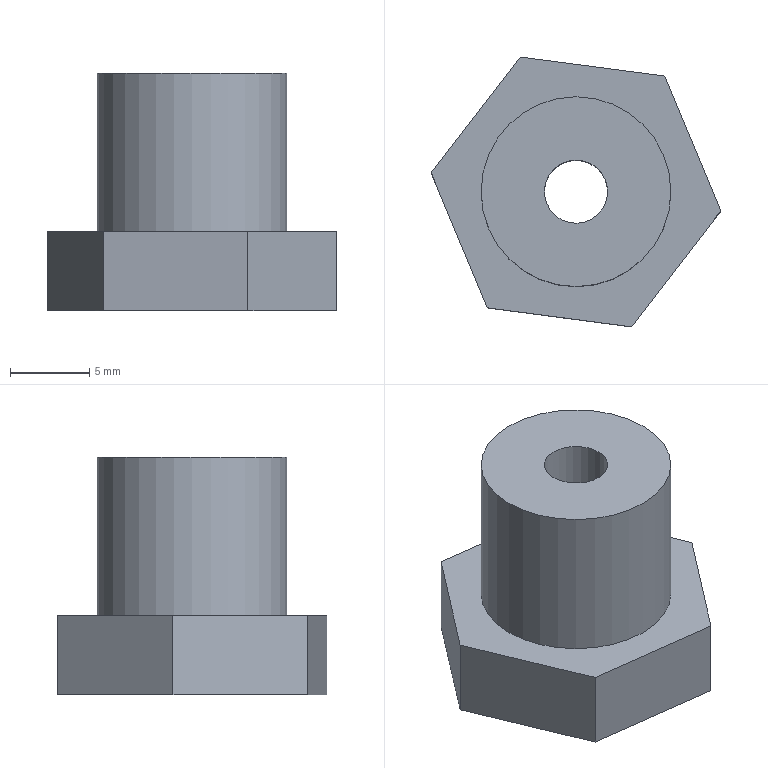Component | NX | 09__27_2 | 1 solid | 11 faces | box 18.32 x 17.07 x 15 mm | volume 2051 mm3 | plane 9 | cylinder 2 | commonest cylinder face diameters 4 x1 12 x1
STEP:
#1=CARTESIAN_POINT('',(0.,0.,0.));
#2=DIRECTION('',(0.,0.,1.));
#3=DIRECTION('',(1.,0.,0.));
#4=AXIS2_PLACEMENT_3D('',#1,#2,#3);
#5=CARTESIAN_POINT('',(70.402,102.259,175.932));
#6=VERTEX_POINT('',#5);
#7=CARTESIAN_POINT('',(66.863,110.792,175.932));
#8=VERTEX_POINT('',#7);
#9=CARTESIAN_POINT('',(70.402,102.259,175.932));
#10=DIRECTION('',(-0.383,0.9237,0.));
#11=VECTOR('',#10,1.);
#12=LINE('',#9,#11);
#13=CARTESIAN_POINT('',(70.402,102.259,170.932));
#14=DIRECTION('',(0.9237,0.383,0.));
#15=DIRECTION('',(0.383,-0.9237,0.));
#16=AXIS2_PLACEMENT_3D('',#13,#14,#15);
#17=PLANE('',#16);
#18=CARTESIAN_POINT('',(0.,-5.));
#19=DIRECTION('',(-1.,0.));
#20=VECTOR('',#19,1.);
#21=LINE('',#18,#20);
#22=(GEOMETRIC_REPRESENTATION_CONTEXT(2)PARAMETRIC_REPRESENTATION_CONTEXT()REPRESENTATION_CONTEXT('',''));
#23=DEFINITIONAL_REPRESENTATION('',(#21),#22);
#24=PCURVE('',#17,#23);
#25=CARTESIAN_POINT('',(76.022,109.59,175.932));
#26=DIRECTION('',(0.,0.,-1.));
#27=DIRECTION('',(0.9237,0.383,0.));
#28=AXIS2_PLACEMENT_3D('',#25,#26,#27);
#29=PLANE('',#28);
#30=CARTESIAN_POINT('',(-8.,4.619));
#31=DIRECTION('',(-0.,-1.));
#32=VECTOR('',#31,1.);
#33=LINE('',#30,#32);
#34=(GEOMETRIC_REPRESENTATION_CONTEXT(2)PARAMETRIC_REPRESENTATION_CONTEXT()REPRESENTATION_CONTEXT('',''));
#35=DEFINITIONAL_REPRESENTATION('',(#33),#34);
#36=PCURVE('',#29,#35);
#37=SURFACE_CURVE('',#12,(#24,#36),.PCURVE_S1.);
#38=EDGE_CURVE('',#6,#8,#37,.T.);
#39=ORIENTED_EDGE('',*,*,#38,.T.);
#40=CARTESIAN_POINT('',(66.863,110.792,170.932));
#41=VERTEX_POINT('',#40);
#42=CARTESIAN_POINT('',(66.863,110.792,170.932));
#43=DIRECTION('',(0.,0.,1.));
#44=VECTOR('',#43,1.);
#45=LINE('',#42,#44);
#46=CARTESIAN_POINT('',(-9.238,0.));
#47=DIRECTION('',(0.,-1.));
#48=VECTOR('',#47,1.);
#49=LINE('',#46,#48);
#50=(GEOMETRIC_REPRESENTATION_CONTEXT(2)PARAMETRIC_REPRESENTATION_CONTEXT()REPRESENTATION_CONTEXT('',''));
#51=DEFINITIONAL_REPRESENTATION('',(#49),#50);
#52=PCURVE('',#17,#51);
#53=CARTESIAN_POINT('',(66.863,110.792,170.932));
#54=DIRECTION('',(0.7936,-0.6084,0.));
#55=DIRECTION('',(-0.6084,-0.7936,0.));
#56=AXIS2_PLACEMENT_3D('',#53,#54,#55);
#57=PLANE('',#56);
#58=CARTESIAN_POINT('',(0.,0.));
#59=DIRECTION('',(0.,-1.));
#60=VECTOR('',#59,1.);
#61=LINE('',#58,#60);
#62=(GEOMETRIC_REPRESENTATION_CONTEXT(2)PARAMETRIC_REPRESENTATION_CONTEXT()REPRESENTATION_CONTEXT('',''));
#63=DEFINITIONAL_REPRESENTATION('',(#61),#62);
#64=PCURVE('',#57,#63);
#65=SURFACE_CURVE('',#45,(#52,#64),.PCURVE_S1.);
#66=EDGE_CURVE('',#41,#8,#65,.T.);
#67=ORIENTED_EDGE('',*,*,#66,.F.);
#68=CARTESIAN_POINT('',(70.402,102.259,170.932));
#69=VERTEX_POINT('',#68);
#70=CARTESIAN_POINT('',(70.402,102.259,170.932));
#71=DIRECTION('',(-0.383,0.9237,0.));
#72=VECTOR('',#71,1.);
#73=LINE('',#70,#72);
#74=CARTESIAN_POINT('',(0.,0.));
#75=DIRECTION('',(-1.,0.));
#76=VECTOR('',#75,1.);
#77=LINE('',#74,#76);
#78=(GEOMETRIC_REPRESENTATION_CONTEXT(2)PARAMETRIC_REPRESENTATION_CONTEXT()REPRESENTATION_CONTEXT('',''));
#79=DEFINITIONAL_REPRESENTATION('',(#77),#78);
#80=PCURVE('',#17,#79);
#81=CARTESIAN_POINT('',(76.022,109.59,170.932));
#82=DIRECTION('',(0.,0.,-1.));
#83=DIRECTION('',(0.9237,0.383,0.));
#84=AXIS2_PLACEMENT_3D('',#81,#82,#83);
#85=PLANE('',#84);
#86=CARTESIAN_POINT('',(-8.,4.619));
#87=DIRECTION('',(-0.,-1.));
#88=VECTOR('',#87,1.);
#89=LINE('',#86,#88);
#90=(GEOMETRIC_REPRESENTATION_CONTEXT(2)PARAMETRIC_REPRESENTATION_CONTEXT()REPRESENTATION_CONTEXT('',''));
#91=DEFINITIONAL_REPRESENTATION('',(#89),#90);
#92=PCURVE('',#85,#91);
#93=SURFACE_CURVE('',#73,(#80,#92),.PCURVE_S1.);
#94=EDGE_CURVE('',#69,#41,#93,.T.);
#95=ORIENTED_EDGE('',*,*,#94,.F.);
#96=CARTESIAN_POINT('',(70.402,102.259,170.932));
#97=DIRECTION('',(0.,0.,1.));
#98=VECTOR('',#97,1.);
#99=LINE('',#96,#98);
#100=CARTESIAN_POINT('',(0.,0.));
#101=DIRECTION('',(0.,-1.));
#102=VECTOR('',#101,1.);
#103=LINE('',#100,#102);
#104=(GEOMETRIC_REPRESENTATION_CONTEXT(2)PARAMETRIC_REPRESENTATION_CONTEXT()REPRESENTATION_CONTEXT('',''));
#105=DEFINITIONAL_REPRESENTATION('',(#103),#104);
#106=PCURVE('',#17,#105);
#107=CARTESIAN_POINT('',(79.561,101.057,170.932));
#108=DIRECTION('',(0.1301,0.9915,0.));
#109=DIRECTION('',(0.9915,-0.1301,0.));
#110=AXIS2_PLACEMENT_3D('',#107,#108,#109);
#111=PLANE('',#110);
#112=CARTESIAN_POINT('',(-9.238,0.));
#113=DIRECTION('',(0.,-1.));
#114=VECTOR('',#113,1.);
#115=LINE('',#112,#114);
#116=(GEOMETRIC_REPRESENTATION_CONTEXT(2)PARAMETRIC_REPRESENTATION_CONTEXT()REPRESENTATION_CONTEXT('',''));
#117=DEFINITIONAL_REPRESENTATION('',(#115),#116);
#118=PCURVE('',#111,#117);
#119=SURFACE_CURVE('',#99,(#106,#118),.PCURVE_S1.);
#120=EDGE_CURVE('',#69,#6,#119,.T.);
#121=ORIENTED_EDGE('',*,*,#120,.T.);
#122=EDGE_LOOP('',(#39,#67,#95,#121));
#123=FACE_BOUND('',#122,.T.);
#124=ADVANCED_FACE('',(#123),#17,.F.);
#125=CARTESIAN_POINT('',(72.484,118.123,175.932));
#126=VERTEX_POINT('',#125);
#127=CARTESIAN_POINT('',(66.863,110.792,175.932));
#128=DIRECTION('',(0.6084,0.7936,0.));
#129=VECTOR('',#128,1.);
#130=LINE('',#127,#129);
#131=CARTESIAN_POINT('',(0.,-5.));
#132=DIRECTION('',(-1.,0.));
#133=VECTOR('',#132,1.);
#134=LINE('',#131,#133);
#135=(GEOMETRIC_REPRESENTATION_CONTEXT(2)PARAMETRIC_REPRESENTATION_CONTEXT()REPRESENTATION_CONTEXT('',''));
#136=DEFINITIONAL_REPRESENTATION('',(#134),#135);
#137=PCURVE('',#57,#136);
#138=CARTESIAN_POINT('',(-8.,-4.619));
#139=DIRECTION('',(0.866,-0.5));
#140=VECTOR('',#139,1.);
#141=LINE('',#138,#140);
#142=(GEOMETRIC_REPRESENTATION_CONTEXT(2)PARAMETRIC_REPRESENTATION_CONTEXT()REPRESENTATION_CONTEXT('',''));
#143=DEFINITIONAL_REPRESENTATION('',(#141),#142);
#144=PCURVE('',#29,#143);
#145=SURFACE_CURVE('',#130,(#137,#144),.PCURVE_S1.);
#146=EDGE_CURVE('',#8,#126,#145,.T.);
#147=ORIENTED_EDGE('',*,*,#146,.T.);
#148=CARTESIAN_POINT('',(72.484,118.123,170.932));
#149=VERTEX_POINT('',#148);
#150=CARTESIAN_POINT('',(72.484,118.123,170.932));
#151=DIRECTION('',(0.,0.,1.));
#152=VECTOR('',#151,1.);
#153=LINE('',#150,#152);
#154=CARTESIAN_POINT('',(-9.238,0.));
#155=DIRECTION('',(0.,-1.));
#156=VECTOR('',#155,1.);
#157=LINE('',#154,#156);
#158=(GEOMETRIC_REPRESENTATION_CONTEXT(2)PARAMETRIC_REPRESENTATION_CONTEXT()REPRESENTATION_CONTEXT('',''));
#159=DEFINITIONAL_REPRESENTATION('',(#157),#158);
#160=PCURVE('',#57,#159);
#161=CARTESIAN_POINT('',(72.484,118.123,170.932));
#162=DIRECTION('',(-0.1301,-0.9915,0.));
#163=DIRECTION('',(-0.9915,0.1301,0.));
#164=AXIS2_PLACEMENT_3D('',#161,#162,#163);
#165=PLANE('',#164);
#166=CARTESIAN_POINT('',(0.,0.));
#167=DIRECTION('',(0.,-1.));
#168=VECTOR('',#167,1.);
#169=LINE('',#166,#168);
#170=(GEOMETRIC_REPRESENTATION_CONTEXT(2)PARAMETRIC_REPRESENTATION_CONTEXT()REPRESENTATION_CONTEXT('',''));
#171=DEFINITIONAL_REPRESENTATION('',(#169),#170);
#172=PCURVE('',#165,#171);
#173=SURFACE_CURVE('',#153,(#160,#172),.PCURVE_S1.);
#174=EDGE_CURVE('',#149,#126,#173,.T.);
#175=ORIENTED_EDGE('',*,*,#174,.F.);
#176=CARTESIAN_POINT('',(66.863,110.792,170.932));
#177=DIRECTION('',(0.6084,0.7936,0.));
#178=VECTOR('',#177,1.);
#179=LINE('',#176,#178);
#180=CARTESIAN_POINT('',(0.,0.));
#181=DIRECTION('',(-1.,0.));
#182=VECTOR('',#181,1.);
#183=LINE('',#180,#182);
#184=(GEOMETRIC_REPRESENTATION_CONTEXT(2)PARAMETRIC_REPRESENTATION_CONTEXT()REPRESENTATION_CONTEXT('',''));
#185=DEFINITIONAL_REPRESENTATION('',(#183),#184);
#186=PCURVE('',#57,#185);
#187=CARTESIAN_POINT('',(-8.,-4.619));
#188=DIRECTION('',(0.866,-0.5));
#189=VECTOR('',#188,1.);
#190=LINE('',#187,#189);
#191=(GEOMETRIC_REPRESENTATION_CONTEXT(2)PARAMETRIC_REPRESENTATION_CONTEXT()REPRESENTATION_CONTEXT('',''));
#192=DEFINITIONAL_REPRESENTATION('',(#190),#191);
#193=PCURVE('',#85,#192);
#194=SURFACE_CURVE('',#179,(#186,#193),.PCURVE_S1.);
#195=EDGE_CURVE('',#41,#149,#194,.T.);
#196=ORIENTED_EDGE('',*,*,#195,.F.);
#197=ORIENTED_EDGE('',*,*,#66,.T.);
#198=EDGE_LOOP('',(#147,#175,#196,#197));
#199=FACE_BOUND('',#198,.T.);
#200=ADVANCED_FACE('',(#199),#57,.F.);
#201=CARTESIAN_POINT('',(81.643,116.921,175.932));
#202=VERTEX_POINT('',#201);
#203=CARTESIAN_POINT('',(72.484,118.123,175.932));
#204=DIRECTION('',(0.9915,-0.1301,0.));
#205=VECTOR('',#204,1.);
#206=LINE('',#203,#205);
#207=CARTESIAN_POINT('',(0.,-5.));
#208=DIRECTION('',(-1.,0.));
#209=VECTOR('',#208,1.);
#210=LINE('',#207,#209);
#211=(GEOMETRIC_REPRESENTATION_CONTEXT(2)PARAMETRIC_REPRESENTATION_CONTEXT()REPRESENTATION_CONTEXT('',''));
#212=DEFINITIONAL_REPRESENTATION('',(#210),#211);
#213=PCURVE('',#165,#212);
#214=CARTESIAN_POINT('',(0.,-9.238));
#215=DIRECTION('',(0.866,0.5));
#216=VECTOR('',#215,1.);
#217=LINE('',#214,#216);
#218=(GEOMETRIC_REPRESENTATION_CONTEXT(2)PARAMETRIC_REPRESENTATION_CONTEXT()REPRESENTATION_CONTEXT('',''));
#219=DEFINITIONAL_REPRESENTATION('',(#217),#218);
#220=PCURVE('',#29,#219);
#221=SURFACE_CURVE('',#206,(#213,#220),.PCURVE_S1.);
#222=EDGE_CURVE('',#126,#202,#221,.T.);
#223=ORIENTED_EDGE('',*,*,#222,.T.);
#224=CARTESIAN_POINT('',(81.643,116.921,170.932));
#225=VERTEX_POINT('',#224);
#226=CARTESIAN_POINT('',(81.643,116.921,170.932));
#227=DIRECTION('',(0.,0.,1.));
#228=VECTOR('',#227,1.);
#229=LINE('',#226,#228);
#230=CARTESIAN_POINT('',(-9.238,0.));
#231=DIRECTION('',(0.,-1.));
#232=VECTOR('',#231,1.);
#233=LINE('',#230,#232);
#234=(GEOMETRIC_REPRESENTATION_CONTEXT(2)PARAMETRIC_REPRESENTATION_CONTEXT()REPRESENTATION_CONTEXT('',''));
#235=DEFINITIONAL_REPRESENTATION('',(#233),#234);
#236=PCURVE('',#165,#235);
#237=CARTESIAN_POINT('',(81.643,116.921,170.932));
#238=DIRECTION('',(-0.9237,-0.383,0.));
#239=DIRECTION('',(-0.383,0.9237,0.));
#240=AXIS2_PLACEMENT_3D('',#237,#238,#239);
#241=PLANE('',#240);
#242=CARTESIAN_POINT('',(0.,0.));
#243=DIRECTION('',(0.,-1.));
#244=VECTOR('',#243,1.);
#245=LINE('',#242,#244);
#246=(GEOMETRIC_REPRESENTATION_CONTEXT(2)PARAMETRIC_REPRESENTATION_CONTEXT()REPRESENTATION_CONTEXT('',''));
#247=DEFINITIONAL_REPRESENTATION('',(#245),#246);
#248=PCURVE('',#241,#247);
#249=SURFACE_CURVE('',#229,(#236,#248),.PCURVE_S1.);
#250=EDGE_CURVE('',#225,#202,#249,.T.);
#251=ORIENTED_EDGE('',*,*,#250,.F.);
#252=CARTESIAN_POINT('',(72.484,118.123,170.932));
#253=DIRECTION('',(0.9915,-0.1301,0.));
#254=VECTOR('',#253,1.);
#255=LINE('',#252,#254);
#256=CARTESIAN_POINT('',(0.,0.));
#257=DIRECTION('',(-1.,0.));
#258=VECTOR('',#257,1.);
#259=LINE('',#256,#258);
#260=(GEOMETRIC_REPRESENTATION_CONTEXT(2)PARAMETRIC_REPRESENTATION_CONTEXT()REPRESENTATION_CONTEXT('',''));
#261=DEFINITIONAL_REPRESENTATION('',(#259),#260);
#262=PCURVE('',#165,#261);
#263=CARTESIAN_POINT('',(0.,-9.238));
#264=DIRECTION('',(0.866,0.5));
#265=VECTOR('',#264,1.);
#266=LINE('',#263,#265);
#267=(GEOMETRIC_REPRESENTATION_CONTEXT(2)PARAMETRIC_REPRESENTATION_CONTEXT()REPRESENTATION_CONTEXT('',''));
#268=DEFINITIONAL_REPRESENTATION('',(#266),#267);
#269=PCURVE('',#85,#268);
#270=SURFACE_CURVE('',#255,(#262,#269),.PCURVE_S1.);
#271=EDGE_CURVE('',#149,#225,#270,.T.);
#272=ORIENTED_EDGE('',*,*,#271,.F.);
#273=ORIENTED_EDGE('',*,*,#174,.T.);
#274=EDGE_LOOP('',(#223,#251,#272,#273));
#275=FACE_BOUND('',#274,.T.);
#276=ADVANCED_FACE('',(#275),#165,.F.);
#277=CARTESIAN_POINT('',(85.181,108.388,175.932));
#278=VERTEX_POINT('',#277);
#279=CARTESIAN_POINT('',(81.643,116.921,175.932));
#280=DIRECTION('',(0.383,-0.9237,0.));
#281=VECTOR('',#280,1.);
#282=LINE('',#279,#281);
#283=CARTESIAN_POINT('',(0.,-5.));
#284=DIRECTION('',(-1.,0.));
#285=VECTOR('',#284,1.);
#286=LINE('',#283,#285);
#287=(GEOMETRIC_REPRESENTATION_CONTEXT(2)PARAMETRIC_REPRESENTATION_CONTEXT()REPRESENTATION_CONTEXT('',''));
#288=DEFINITIONAL_REPRESENTATION('',(#286),#287);
#289=PCURVE('',#241,#288);
#290=CARTESIAN_POINT('',(8.,-4.619));
#291=DIRECTION('',(0.,1.));
#292=VECTOR('',#291,1.);
#293=LINE('',#290,#292);
#294=(GEOMETRIC_REPRESENTATION_CONTEXT(2)PARAMETRIC_REPRESENTATION_CONTEXT()REPRESENTATION_CONTEXT('',''));
#295=DEFINITIONAL_REPRESENTATION('',(#293),#294);
#296=PCURVE('',#29,#295);
#297=SURFACE_CURVE('',#282,(#289,#296),.PCURVE_S1.);
#298=EDGE_CURVE('',#202,#278,#297,.T.);
#299=ORIENTED_EDGE('',*,*,#298,.T.);
#300=CARTESIAN_POINT('',(85.181,108.388,170.932));
#301=VERTEX_POINT('',#300);
#302=CARTESIAN_POINT('',(85.181,108.388,170.932));
#303=DIRECTION('',(0.,0.,1.));
#304=VECTOR('',#303,1.);
#305=LINE('',#302,#304);
#306=CARTESIAN_POINT('',(-9.238,0.));
#307=DIRECTION('',(0.,-1.));
#308=VECTOR('',#307,1.);
#309=LINE('',#306,#308);
#310=(GEOMETRIC_REPRESENTATION_CONTEXT(2)PARAMETRIC_REPRESENTATION_CONTEXT()REPRESENTATION_CONTEXT('',''));
#311=DEFINITIONAL_REPRESENTATION('',(#309),#310);
#312=PCURVE('',#241,#311);
#313=CARTESIAN_POINT('',(85.181,108.388,170.932));
#314=DIRECTION('',(-0.7936,0.6084,0.));
#315=DIRECTION('',(0.6084,0.7936,0.));
#316=AXIS2_PLACEMENT_3D('',#313,#314,#315);
#317=PLANE('',#316);
#318=CARTESIAN_POINT('',(0.,0.));
#319=DIRECTION('',(0.,-1.));
#320=VECTOR('',#319,1.);
#321=LINE('',#318,#320);
#322=(GEOMETRIC_REPRESENTATION_CONTEXT(2)PARAMETRIC_REPRESENTATION_CONTEXT()REPRESENTATION_CONTEXT('',''));
#323=DEFINITIONAL_REPRESENTATION('',(#321),#322);
#324=PCURVE('',#317,#323);
#325=SURFACE_CURVE('',#305,(#312,#324),.PCURVE_S1.);
#326=EDGE_CURVE('',#301,#278,#325,.T.);
#327=ORIENTED_EDGE('',*,*,#326,.F.);
#328=CARTESIAN_POINT('',(81.643,116.921,170.932));
#329=DIRECTION('',(0.383,-0.9237,0.));
#330=VECTOR('',#329,1.);
#331=LINE('',#328,#330);
#332=CARTESIAN_POINT('',(0.,0.));
#333=DIRECTION('',(-1.,0.));
#334=VECTOR('',#333,1.);
#335=LINE('',#332,#334);
#336=(GEOMETRIC_REPRESENTATION_CONTEXT(2)PARAMETRIC_REPRESENTATION_CONTEXT()REPRESENTATION_CONTEXT('',''));
#337=DEFINITIONAL_REPRESENTATION('',(#335),#336);
#338=PCURVE('',#241,#337);
#339=CARTESIAN_POINT('',(8.,-4.619));
#340=DIRECTION('',(0.,1.));
#341=VECTOR('',#340,1.);
#342=LINE('',#339,#341);
#343=(GEOMETRIC_REPRESENTATION_CONTEXT(2)PARAMETRIC_REPRESENTATION_CONTEXT()REPRESENTATION_CONTEXT('',''));
#344=DEFINITIONAL_REPRESENTATION('',(#342),#343);
#345=PCURVE('',#85,#344);
#346=SURFACE_CURVE('',#331,(#338,#345),.PCURVE_S1.);
#347=EDGE_CURVE('',#225,#301,#346,.T.);
#348=ORIENTED_EDGE('',*,*,#347,.F.);
#349=ORIENTED_EDGE('',*,*,#250,.T.);
#350=EDGE_LOOP('',(#299,#327,#348,#349));
#351=FACE_BOUND('',#350,.T.);
#352=ADVANCED_FACE('',(#351),#241,.F.);
#353=CARTESIAN_POINT('',(79.561,101.057,175.932));
#354=VERTEX_POINT('',#353);
#355=CARTESIAN_POINT('',(85.181,108.388,175.932));
#356=DIRECTION('',(-0.6084,-0.7936,0.));
#357=VECTOR('',#356,1.);
#358=LINE('',#355,#357);
#359=CARTESIAN_POINT('',(0.,-5.));
#360=DIRECTION('',(-1.,0.));
#361=VECTOR('',#360,1.);
#362=LINE('',#359,#361);
#363=(GEOMETRIC_REPRESENTATION_CONTEXT(2)PARAMETRIC_REPRESENTATION_CONTEXT()REPRESENTATION_CONTEXT('',''));
#364=DEFINITIONAL_REPRESENTATION('',(#362),#363);
#365=PCURVE('',#317,#364);
#366=CARTESIAN_POINT('',(8.,4.619));
#367=DIRECTION('',(-0.866,0.5));
#368=VECTOR('',#367,1.);
#369=LINE('',#366,#368);
#370=(GEOMETRIC_REPRESENTATION_CONTEXT(2)PARAMETRIC_REPRESENTATION_CONTEXT()REPRESENTATION_CONTEXT('',''));
#371=DEFINITIONAL_REPRESENTATION('',(#369),#370);
#372=PCURVE('',#29,#371);
#373=SURFACE_CURVE('',#358,(#365,#372),.PCURVE_S1.);
#374=EDGE_CURVE('',#278,#354,#373,.T.);
#375=ORIENTED_EDGE('',*,*,#374,.T.);
#376=CARTESIAN_POINT('',(79.561,101.057,170.932));
#377=VERTEX_POINT('',#376);
#378=CARTESIAN_POINT('',(79.561,101.057,170.932));
#379=DIRECTION('',(0.,0.,1.));
#380=VECTOR('',#379,1.);
#381=LINE('',#378,#380);
#382=CARTESIAN_POINT('',(-9.238,0.));
#383=DIRECTION('',(0.,-1.));
#384=VECTOR('',#383,1.);
#385=LINE('',#382,#384);
#386=(GEOMETRIC_REPRESENTATION_CONTEXT(2)PARAMETRIC_REPRESENTATION_CONTEXT()REPRESENTATION_CONTEXT('',''));
#387=DEFINITIONAL_REPRESENTATION('',(#385),#386);
#388=PCURVE('',#317,#387);
#389=CARTESIAN_POINT('',(0.,0.));
#390=DIRECTION('',(0.,-1.));
#391=VECTOR('',#390,1.);
#392=LINE('',#389,#391);
#393=(GEOMETRIC_REPRESENTATION_CONTEXT(2)PARAMETRIC_REPRESENTATION_CONTEXT()REPRESENTATION_CONTEXT('',''));
#394=DEFINITIONAL_REPRESENTATION('',(#392),#393);
#395=PCURVE('',#111,#394);
#396=SURFACE_CURVE('',#381,(#388,#395),.PCURVE_S1.);
#397=EDGE_CURVE('',#377,#354,#396,.T.);
#398=ORIENTED_EDGE('',*,*,#397,.F.);
#399=CARTESIAN_POINT('',(85.181,108.388,170.932));
#400=DIRECTION('',(-0.6084,-0.7936,0.));
#401=VECTOR('',#400,1.);
#402=LINE('',#399,#401);
#403=CARTESIAN_POINT('',(0.,0.));
#404=DIRECTION('',(-1.,0.));
#405=VECTOR('',#404,1.);
#406=LINE('',#403,#405);
#407=(GEOMETRIC_REPRESENTATION_CONTEXT(2)PARAMETRIC_REPRESENTATION_CONTEXT()REPRESENTATION_CONTEXT('',''));
#408=DEFINITIONAL_REPRESENTATION('',(#406),#407);
#409=PCURVE('',#317,#408);
#410=CARTESIAN_POINT('',(8.,4.619));
#411=DIRECTION('',(-0.866,0.5));
#412=VECTOR('',#411,1.);
#413=LINE('',#410,#412);
#414=(GEOMETRIC_REPRESENTATION_CONTEXT(2)PARAMETRIC_REPRESENTATION_CONTEXT()REPRESENTATION_CONTEXT('',''));
#415=DEFINITIONAL_REPRESENTATION('',(#413),#414);
#416=PCURVE('',#85,#415);
#417=SURFACE_CURVE('',#402,(#409,#416),.PCURVE_S1.);
#418=EDGE_CURVE('',#301,#377,#417,.T.);
#419=ORIENTED_EDGE('',*,*,#418,.F.);
#420=ORIENTED_EDGE('',*,*,#326,.T.);
#421=EDGE_LOOP('',(#375,#398,#419,#420));
#422=FACE_BOUND('',#421,.T.);
#423=ADVANCED_FACE('',(#422),#317,.F.);
#424=CARTESIAN_POINT('',(79.561,101.057,175.932));
#425=DIRECTION('',(-0.9915,0.1301,0.));
#426=VECTOR('',#425,1.);
#427=LINE('',#424,#426);
#428=CARTESIAN_POINT('',(0.,-5.));
#429=DIRECTION('',(-1.,0.));
#430=VECTOR('',#429,1.);
#431=LINE('',#428,#430);
#432=(GEOMETRIC_REPRESENTATION_CONTEXT(2)PARAMETRIC_REPRESENTATION_CONTEXT()REPRESENTATION_CONTEXT('',''));
#433=DEFINITIONAL_REPRESENTATION('',(#431),#432);
#434=PCURVE('',#111,#433);
#435=CARTESIAN_POINT('',(-0.,9.238));
#436=DIRECTION('',(-0.866,-0.5));
#437=VECTOR('',#436,1.);
#438=LINE('',#435,#437);
#439=(GEOMETRIC_REPRESENTATION_CONTEXT(2)PARAMETRIC_REPRESENTATION_CONTEXT()REPRESENTATION_CONTEXT('',''));
#440=DEFINITIONAL_REPRESENTATION('',(#438),#439);
#441=PCURVE('',#29,#440);
#442=SURFACE_CURVE('',#427,(#434,#441),.PCURVE_S1.);
#443=EDGE_CURVE('',#354,#6,#442,.T.);
#444=ORIENTED_EDGE('',*,*,#443,.T.);
#445=ORIENTED_EDGE('',*,*,#120,.F.);
#446=CARTESIAN_POINT('',(79.561,101.057,170.932));
#447=DIRECTION('',(-0.9915,0.1301,0.));
#448=VECTOR('',#447,1.);
#449=LINE('',#446,#448);
#450=CARTESIAN_POINT('',(0.,0.));
#451=DIRECTION('',(-1.,0.));
#452=VECTOR('',#451,1.);
#453=LINE('',#450,#452);
#454=(GEOMETRIC_REPRESENTATION_CONTEXT(2)PARAMETRIC_REPRESENTATION_CONTEXT()REPRESENTATION_CONTEXT('',''));
#455=DEFINITIONAL_REPRESENTATION('',(#453),#454);
#456=PCURVE('',#111,#455);
#457=CARTESIAN_POINT('',(-0.,9.238));
#458=DIRECTION('',(-0.866,-0.5));
#459=VECTOR('',#458,1.);
#460=LINE('',#457,#459);
#461=(GEOMETRIC_REPRESENTATION_CONTEXT(2)PARAMETRIC_REPRESENTATION_CONTEXT()REPRESENTATION_CONTEXT('',''));
#462=DEFINITIONAL_REPRESENTATION('',(#460),#461);
#463=PCURVE('',#85,#462);
#464=SURFACE_CURVE('',#449,(#456,#463),.PCURVE_S1.);
#465=EDGE_CURVE('',#377,#69,#464,.T.);
#466=ORIENTED_EDGE('',*,*,#465,.F.);
#467=ORIENTED_EDGE('',*,*,#397,.T.);
#468=EDGE_LOOP('',(#444,#445,#466,#467));
#469=FACE_BOUND('',#468,.T.);
#470=ADVANCED_FACE('',(#469),#111,.F.);
#471=CARTESIAN_POINT('',(77.87,110.356,170.932));
#472=VERTEX_POINT('',#471);
#473=CARTESIAN_POINT('',(76.022,109.59,170.932));
#474=DIRECTION('',(0.,0.,-1.));
#475=DIRECTION('',(0.9237,0.383,0.));
#476=AXIS2_PLACEMENT_3D('',#473,#474,#475);
#477=CIRCLE('',#476,2.);
#478=CARTESIAN_POINT('',(76.022,109.59,170.932));
#479=DIRECTION('',(0.,0.,1.));
#480=DIRECTION('',(-0.9237,-0.383,0.));
#481=AXIS2_PLACEMENT_3D('',#478,#479,#480);
#482=CYLINDRICAL_SURFACE('',#481,2.);
#483=CARTESIAN_POINT('',(9.425,0.));
#484=DIRECTION('',(-1.,0.));
#485=VECTOR('',#484,1.);
#486=LINE('',#483,#485);
#487=(GEOMETRIC_REPRESENTATION_CONTEXT(2)PARAMETRIC_REPRESENTATION_CONTEXT()REPRESENTATION_CONTEXT('',''));
#488=DEFINITIONAL_REPRESENTATION('',(#486),#487);
#489=PCURVE('',#482,#488);
#490=CARTESIAN_POINT('',(0.,0.));
#491=DIRECTION('',(1.,-0.));
#492=AXIS2_PLACEMENT_2D('',#490,#491);
#493=CIRCLE('',#492,2.);
#494=(GEOMETRIC_REPRESENTATION_CONTEXT(2)PARAMETRIC_REPRESENTATION_CONTEXT()REPRESENTATION_CONTEXT('',''));
#495=DEFINITIONAL_REPRESENTATION('',(#493),#494);
#496=PCURVE('',#85,#495);
#497=SURFACE_CURVE('',#477,(#489,#496),.PCURVE_S1.);
#498=EDGE_CURVE('',#472,#472,#497,.T.);
#499=ORIENTED_EDGE('',*,*,#498,.F.);
#500=CARTESIAN_POINT('',(77.87,110.356,185.932));
#501=VERTEX_POINT('',#500);
#502=CARTESIAN_POINT('',(77.87,110.356,170.932));
#503=CARTESIAN_POINT('',(77.87,110.356,185.932));
#504=B_SPLINE_CURVE_WITH_KNOTS('',1,(#502,#503),.UNSPECIFIED.,.F.,.F.,(2,2),(0.,15.),.PIECEWISE_BEZIER_KNOTS.);
#505=CARTESIAN_POINT('',(9.425,0.));
#506=DIRECTION('',(0.,1.));
#507=VECTOR('',#506,1.);
#508=LINE('',#505,#507);
#509=(GEOMETRIC_REPRESENTATION_CONTEXT(2)PARAMETRIC_REPRESENTATION_CONTEXT()REPRESENTATION_CONTEXT('',''));
#510=DEFINITIONAL_REPRESENTATION('',(#508),#509);
#511=PCURVE('',#482,#510);
#512=CARTESIAN_POINT('',(3.142,0.));
#513=DIRECTION('',(0.,1.));
#514=VECTOR('',#513,1.);
#515=LINE('',#512,#514);
#516=(GEOMETRIC_REPRESENTATION_CONTEXT(2)PARAMETRIC_REPRESENTATION_CONTEXT()REPRESENTATION_CONTEXT('',''));
#517=DEFINITIONAL_REPRESENTATION('',(#515),#516);
#518=PCURVE('',#482,#517);
#519=SEAM_CURVE('',#504,(#511,#518),.PCURVE_S1.);
#520=EDGE_CURVE('',#472,#501,#519,.T.);
#521=ORIENTED_EDGE('',*,*,#520,.T.);
#522=CARTESIAN_POINT('',(76.022,109.59,185.932));
#523=DIRECTION('',(0.,0.,-1.));
#524=DIRECTION('',(0.9237,0.383,0.));
#525=AXIS2_PLACEMENT_3D('',#522,#523,#524);
#526=CIRCLE('',#525,2.);
#527=CARTESIAN_POINT('',(9.425,15.));
#528=DIRECTION('',(-1.,0.));
#529=VECTOR('',#528,1.);
#530=LINE('',#527,#529);
#531=(GEOMETRIC_REPRESENTATION_CONTEXT(2)PARAMETRIC_REPRESENTATION_CONTEXT()REPRESENTATION_CONTEXT('',''));
#532=DEFINITIONAL_REPRESENTATION('',(#530),#531);
#533=PCURVE('',#482,#532);
#534=CARTESIAN_POINT('',(76.022,109.59,185.932));
#535=DIRECTION('',(0.,0.,-1.));
#536=DIRECTION('',(0.9237,0.383,0.));
#537=AXIS2_PLACEMENT_3D('',#534,#535,#536);
#538=PLANE('',#537);
#539=CARTESIAN_POINT('',(0.,0.));
#540=DIRECTION('',(1.,-0.));
#541=AXIS2_PLACEMENT_2D('',#539,#540);
#542=CIRCLE('',#541,2.);
#543=(GEOMETRIC_REPRESENTATION_CONTEXT(2)PARAMETRIC_REPRESENTATION_CONTEXT()REPRESENTATION_CONTEXT('',''));
#544=DEFINITIONAL_REPRESENTATION('',(#542),#543);
#545=PCURVE('',#538,#544);
#546=SURFACE_CURVE('',#526,(#533,#545),.PCURVE_S1.);
#547=EDGE_CURVE('',#501,#501,#546,.T.);
#548=ORIENTED_EDGE('',*,*,#547,.T.);
#549=ORIENTED_EDGE('',*,*,#520,.F.);
#550=EDGE_LOOP('',(#499,#521,#548,#549));
#551=FACE_BOUND('',#550,.F.);
#552=ADVANCED_FACE('',(#551),#482,.F.);
#553=ORIENTED_EDGE('',*,*,#94,.T.);
#554=ORIENTED_EDGE('',*,*,#195,.T.);
#555=ORIENTED_EDGE('',*,*,#271,.T.);
#556=ORIENTED_EDGE('',*,*,#347,.T.);
#557=ORIENTED_EDGE('',*,*,#418,.T.);
#558=ORIENTED_EDGE('',*,*,#465,.T.);
#559=EDGE_LOOP('',(#553,#554,#555,#556,#557,#558));
#560=FACE_BOUND('',#559,.T.);
#561=ORIENTED_EDGE('',*,*,#498,.F.);
#562=EDGE_LOOP('',(#561));
#563=FACE_BOUND('',#562,.T.);
#564=ADVANCED_FACE('',(#560,#563),#85,.T.);
#565=CARTESIAN_POINT('',(81.565,111.888,175.932));
#566=VERTEX_POINT('',#565);
#567=CARTESIAN_POINT('',(76.022,109.59,175.932));
#568=DIRECTION('',(0.,0.,-1.));
#569=DIRECTION('',(0.9237,0.383,0.));
#570=AXIS2_PLACEMENT_3D('',#567,#568,#569);
#571=CIRCLE('',#570,6.);
#572=CARTESIAN_POINT('',(0.,0.));
#573=DIRECTION('',(1.,0.));
#574=AXIS2_PLACEMENT_2D('',#572,#573);
#575=CIRCLE('',#574,6.);
#576=(GEOMETRIC_REPRESENTATION_CONTEXT(2)PARAMETRIC_REPRESENTATION_CONTEXT()REPRESENTATION_CONTEXT('',''));
#577=DEFINITIONAL_REPRESENTATION('',(#575),#576);
#578=PCURVE('',#29,#577);
#579=CARTESIAN_POINT('',(76.022,109.59,185.932));
#580=DIRECTION('',(0.,0.,-1.));
#581=DIRECTION('',(0.9237,0.383,0.));
#582=AXIS2_PLACEMENT_3D('',#579,#580,#581);
#583=CYLINDRICAL_SURFACE('',#582,6.);
#584=CARTESIAN_POINT('',(0.,10.));
#585=DIRECTION('',(1.,0.));
#586=VECTOR('',#585,1.);
#587=LINE('',#584,#586);
#588=(GEOMETRIC_REPRESENTATION_CONTEXT(2)PARAMETRIC_REPRESENTATION_CONTEXT()REPRESENTATION_CONTEXT('',''));
#589=DEFINITIONAL_REPRESENTATION('',(#587),#588);
#590=PCURVE('',#583,#589);
#591=SURFACE_CURVE('',#571,(#578,#590),.PCURVE_S1.);
#592=EDGE_CURVE('',#566,#566,#591,.T.);
#593=ORIENTED_EDGE('',*,*,#592,.T.);
#594=EDGE_LOOP('',(#593));
#595=FACE_BOUND('',#594,.T.);
#596=ORIENTED_EDGE('',*,*,#38,.F.);
#597=ORIENTED_EDGE('',*,*,#443,.F.);
#598=ORIENTED_EDGE('',*,*,#374,.F.);
#599=ORIENTED_EDGE('',*,*,#298,.F.);
#600=ORIENTED_EDGE('',*,*,#222,.F.);
#601=ORIENTED_EDGE('',*,*,#146,.F.);
#602=EDGE_LOOP('',(#596,#597,#598,#599,#600,#601));
#603=FACE_BOUND('',#602,.T.);
#604=ADVANCED_FACE('',(#595,#603),#29,.F.);
#605=CARTESIAN_POINT('',(81.565,111.888,185.932));
#606=VERTEX_POINT('',#605);
#607=CARTESIAN_POINT('',(76.022,109.59,185.932));
#608=DIRECTION('',(0.,0.,-1.));
#609=DIRECTION('',(0.9237,0.383,0.));
#610=AXIS2_PLACEMENT_3D('',#607,#608,#609);
#611=CIRCLE('',#610,6.);
#612=CARTESIAN_POINT('',(0.,0.));
#613=DIRECTION('',(1.,0.));
#614=VECTOR('',#613,1.);
#615=LINE('',#612,#614);
#616=(GEOMETRIC_REPRESENTATION_CONTEXT(2)PARAMETRIC_REPRESENTATION_CONTEXT()REPRESENTATION_CONTEXT('',''));
#617=DEFINITIONAL_REPRESENTATION('',(#615),#616);
#618=PCURVE('',#583,#617);
#619=CARTESIAN_POINT('',(0.,0.));
#620=DIRECTION('',(1.,0.));
#621=AXIS2_PLACEMENT_2D('',#619,#620);
#622=CIRCLE('',#621,6.);
#623=(GEOMETRIC_REPRESENTATION_CONTEXT(2)PARAMETRIC_REPRESENTATION_CONTEXT()REPRESENTATION_CONTEXT('',''));
#624=DEFINITIONAL_REPRESENTATION('',(#622),#623);
#625=PCURVE('',#538,#624);
#626=SURFACE_CURVE('',#611,(#618,#625),.PCURVE_S1.);
#627=EDGE_CURVE('',#606,#606,#626,.T.);
#628=ORIENTED_EDGE('',*,*,#627,.T.);
#629=CARTESIAN_POINT('',(81.565,111.888,185.932));
#630=CARTESIAN_POINT('',(81.565,111.888,175.932));
#631=B_SPLINE_CURVE_WITH_KNOTS('',1,(#629,#630),.UNSPECIFIED.,.F.,.F.,(2,2),(0.,10.),.PIECEWISE_BEZIER_KNOTS.);
#632=CARTESIAN_POINT('',(6.283,0.));
#633=DIRECTION('',(0.,1.));
#634=VECTOR('',#633,1.);
#635=LINE('',#632,#634);
#636=(GEOMETRIC_REPRESENTATION_CONTEXT(2)PARAMETRIC_REPRESENTATION_CONTEXT()REPRESENTATION_CONTEXT('',''));
#637=DEFINITIONAL_REPRESENTATION('',(#635),#636);
#638=PCURVE('',#583,#637);
#639=CARTESIAN_POINT('',(0.,0.));
#640=DIRECTION('',(0.,1.));
#641=VECTOR('',#640,1.);
#642=LINE('',#639,#641);
#643=(GEOMETRIC_REPRESENTATION_CONTEXT(2)PARAMETRIC_REPRESENTATION_CONTEXT()REPRESENTATION_CONTEXT('',''));
#644=DEFINITIONAL_REPRESENTATION('',(#642),#643);
#645=PCURVE('',#583,#644);
#646=SEAM_CURVE('',#631,(#638,#645),.PCURVE_S1.);
#647=EDGE_CURVE('',#606,#566,#646,.T.);
#648=ORIENTED_EDGE('',*,*,#647,.T.);
#649=ORIENTED_EDGE('',*,*,#592,.F.);
#650=ORIENTED_EDGE('',*,*,#647,.F.);
#651=EDGE_LOOP('',(#628,#648,#649,#650));
#652=FACE_BOUND('',#651,.T.);
#653=ADVANCED_FACE('',(#652),#583,.T.);
#654=ORIENTED_EDGE('',*,*,#627,.F.);
#655=EDGE_LOOP('',(#654));
#656=FACE_BOUND('',#655,.T.);
#657=ORIENTED_EDGE('',*,*,#547,.T.);
#658=EDGE_LOOP('',(#657));
#659=FACE_BOUND('',#658,.T.);
#660=ADVANCED_FACE('',(#656,#659),#538,.F.);
#661=CLOSED_SHELL('',(#124,#200,#276,#352,#423,#470,#552,#564,#604,#653,#660));
#662=MANIFOLD_SOLID_BREP('',#661);
#663=(LENGTH_UNIT()NAMED_UNIT(*)SI_UNIT(.MILLI.,.METRE.));
#664=UNCERTAINTY_MEASURE_WITH_UNIT(LENGTH_MEASURE(0.000002),#663,'','');
#665=(NAMED_UNIT(*)PLANE_ANGLE_UNIT()SI_UNIT($,.RADIAN.));
#666=(NAMED_UNIT(*)SI_UNIT($,.STERADIAN.)SOLID_ANGLE_UNIT());
#667=(GEOMETRIC_REPRESENTATION_CONTEXT(3)GLOBAL_UNCERTAINTY_ASSIGNED_CONTEXT((#664))GLOBAL_UNIT_ASSIGNED_CONTEXT((#663,#665,#666))REPRESENTATION_CONTEXT('',''));
#668=ADVANCED_BREP_SHAPE_REPRESENTATION('',(#4,#662),#667);